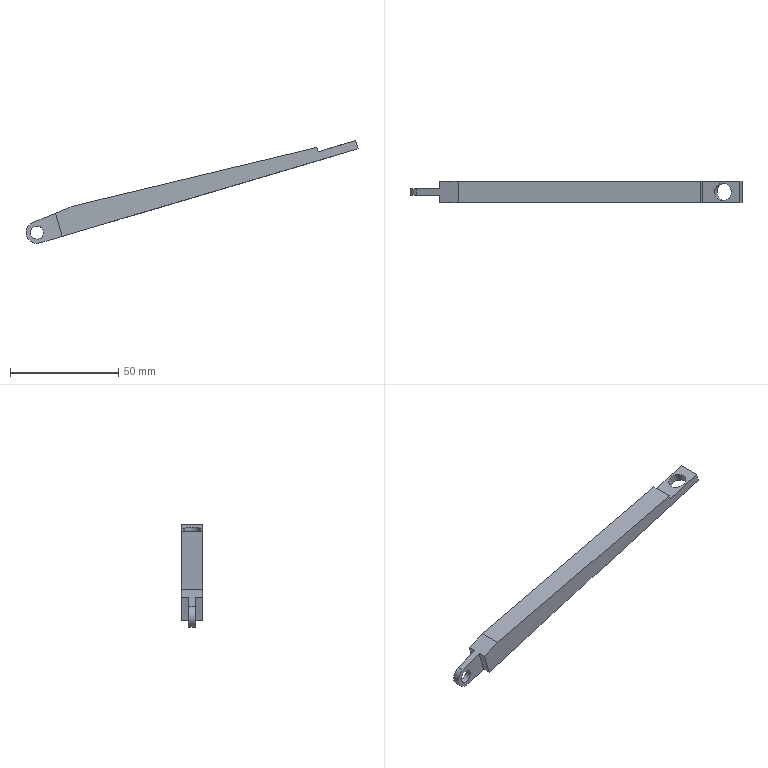Component | NX | LEVER | 1 solid | 17 faces | volume 12238 mm3 | plane 13 | cylinder 3 | sphere 1 | commonest cylinder face diameters 10 x1 6 x1 8 x1